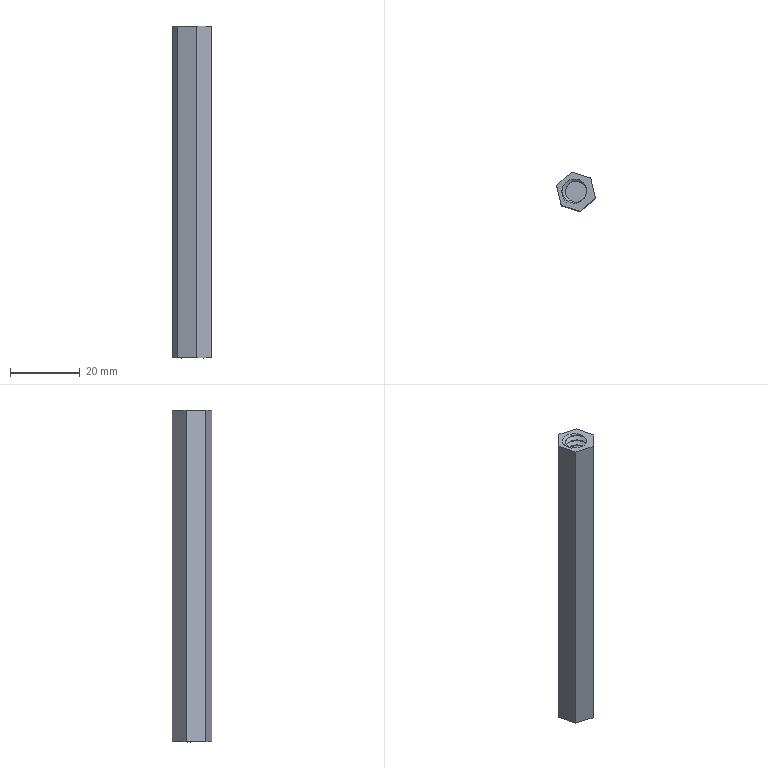Component | SolidWorks | HexRod-1 | 1 solid | 81 faces | volume 6800 mm3 | cylinder 65 | plane 12 | spline 4 | commonest cylinder face diameters 6 x65